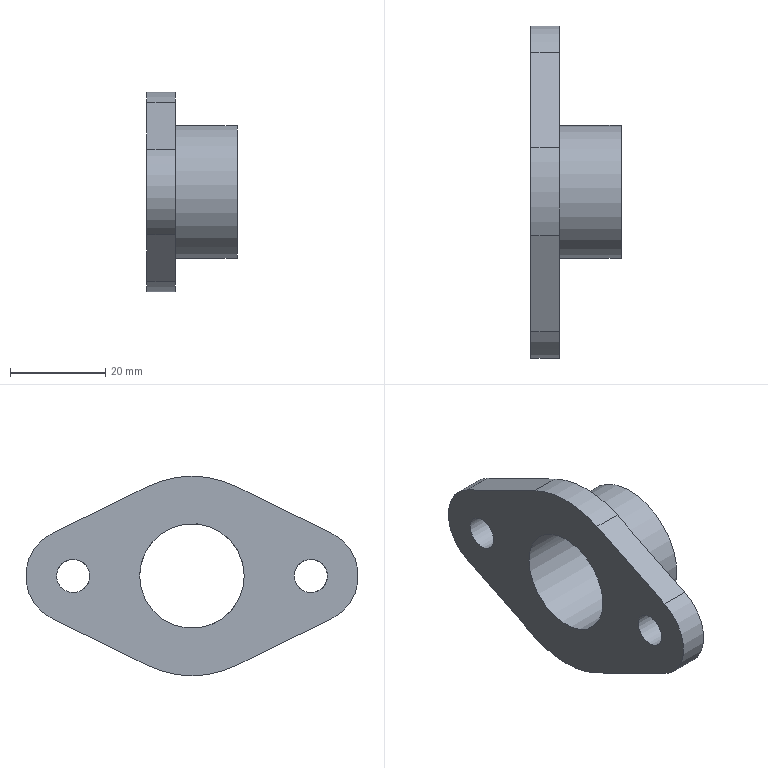Component | NX | PACKING_GLAND | 1 solid | 15 faces | volume 12225 mm3 | cylinder 8 | plane 6 | cone 1 | commonest cylinder face diameters 20 x2 42 x2 7 x2 22 x1 28 x1